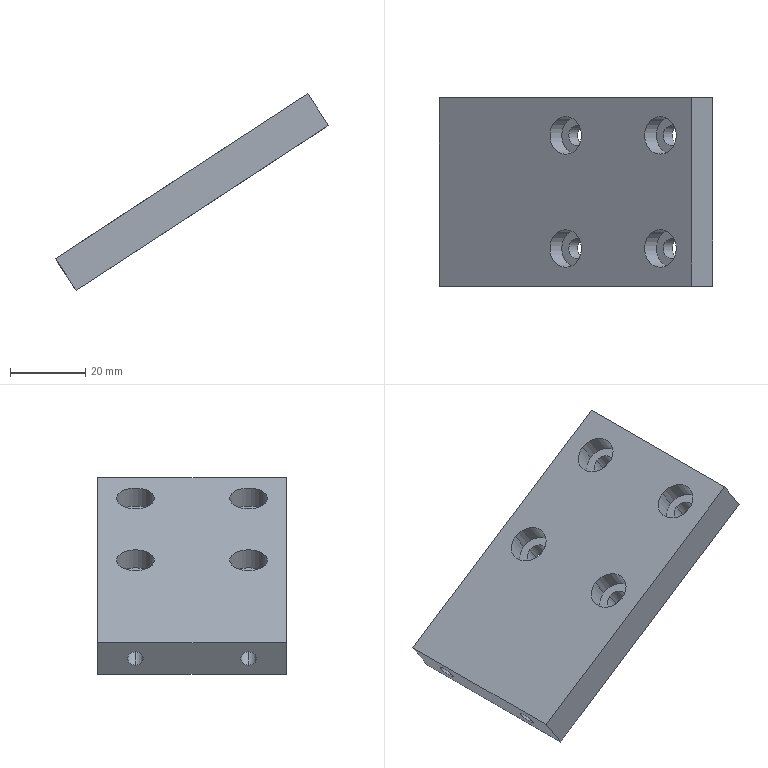Component | SolidWorks | ShimPlate02-1 | 1 solid | 34 faces | box 72.44 x 50 x 52.14 mm | volume 37445 mm3 | cylinder 20 | plane 10 | cone 4 | commonest cylinder face diameters 10 x8 5.5 x8 4.2 x4
build123d program:
from build123d import *

# Parameters (mm, degrees)
SKETCH1_W                                            = 50
SKETCH1_H                                            = 80
BOSS_EXTRUDE1_DEPTH                                  = 10
M5_TAPPED_HOLE1_D                                    = 4.2
M5_TAPPED_HOLE1_DEPTH                                = 12.4
M5_TAPPED_HOLE1_TIP                                  = 1.262
HOLE_SIZE_ACCORDING_TO_THE_TYPE_OF_HEXAG_D           = 5.5
HOLE_SIZE_ACCORDING_TO_THE_TYPE_OF_HEXAG_CBORE_D     = 10
HOLE_SIZE_ACCORDING_TO_THE_TYPE_OF_HEXAG_CBORE_DEPTH = 5.7


with BuildPart() as part:
    # Sketch1 → Boss-Extrude1 (new body)
    with BuildSketch(Plane.XY):
        Rectangle(SKETCH1_W, SKETCH1_H)
    extrude(amount=BOSS_EXTRUDE1_DEPTH)

    # M5 Tapped Hole1
    with Locations(Plane(origin=(0, -40, 0), x_dir=(-1, 0, 0), z_dir=(0, -1, 0))):
        with Locations((15, -5), (-15, -5)):
            Hole(M5_TAPPED_HOLE1_D / 2, depth=M5_TAPPED_HOLE1_DEPTH)
            with Locations((0, 0, -(M5_TAPPED_HOLE1_DEPTH + M5_TAPPED_HOLE1_TIP / 2))):  # 118° drill point
                Cone(0, M5_TAPPED_HOLE1_D / 2, M5_TAPPED_HOLE1_TIP, mode=Mode.SUBTRACT)

    # Hole Size according to the type of hexag (through all)
    with Locations(Plane.XY.offset(10)):
        with Locations((-15, 30), (15, 30), (15, 0), (-15, 0)):
            CounterBoreHole(HOLE_SIZE_ACCORDING_TO_THE_TYPE_OF_HEXAG_D / 2, HOLE_SIZE_ACCORDING_TO_THE_TYPE_OF_HEXAG_CBORE_D / 2, HOLE_SIZE_ACCORDING_TO_THE_TYPE_OF_HEXAG_CBORE_DEPTH)


solid = part.part

# Placed as in the assembly
solid = solid.moved(Location((-58.174, 149.546, 0.7149), (0, -33.165, -90)))
STEP:
#1=COLOUR_RGB('',0.7922,0.8196,0.9333);
#2=FILL_AREA_STYLE_COLOUR('',#1);
#3=FILL_AREA_STYLE('',(#2));
#4=SURFACE_STYLE_FILL_AREA(#3);
#5=SURFACE_SIDE_STYLE('',(#4));
#6=SURFACE_STYLE_USAGE(.BOTH.,#5);
#7=PRESENTATION_STYLE_ASSIGNMENT((#6));
#8=CARTESIAN_POINT('',(-1.394,6.675,0.816));
#9=VERTEX_POINT('',#8);
#10=CARTESIAN_POINT('',(-1.394,6.281,0.816));
#11=VERTEX_POINT('',#10);
#12=CARTESIAN_POINT('',(-1.394,6.478,0.816));
#13=DIRECTION('',(-0.5471,0.,0.8371));
#14=DIRECTION('',(-0.,-1.,0.));
#15=AXIS2_PLACEMENT_3D('',#12,#13,#14);
#16=CIRCLE('',#15,0.1969);
#17=EDGE_CURVE('',#9,#11,#16,.T.);
#18=ORIENTED_EDGE('',*,*,#17,.F.);
#19=CARTESIAN_POINT('',(-1.517,6.675,1.004));
#20=VERTEX_POINT('',#19);
#21=CARTESIAN_POINT('',(-1.517,6.675,1.004));
#22=DIRECTION('',(-0.5471,0.,0.8371));
#23=VECTOR('',#22,39.37);
#24=LINE('',#21,#23);
#25=EDGE_CURVE('',#9,#20,#24,.T.);
#26=ORIENTED_EDGE('',*,*,#25,.T.);
#27=CARTESIAN_POINT('',(-1.517,6.281,1.004));
#28=VERTEX_POINT('',#27);
#29=CARTESIAN_POINT('',(-1.517,6.478,1.004));
#30=DIRECTION('',(-0.5471,0.,0.8371));
#31=DIRECTION('',(-0.,-1.,0.));
#32=AXIS2_PLACEMENT_3D('',#29,#30,#31);
#33=CIRCLE('',#32,0.1969);
#34=EDGE_CURVE('',#20,#28,#33,.T.);
#35=ORIENTED_EDGE('',*,*,#34,.T.);
#36=CARTESIAN_POINT('',(-1.517,6.281,1.004));
#37=DIRECTION('',(-0.5471,0.,0.8371));
#38=VECTOR('',#37,39.37);
#39=LINE('',#36,#38);
#40=EDGE_CURVE('',#11,#28,#39,.T.);
#41=ORIENTED_EDGE('',*,*,#40,.F.);
#42=EDGE_LOOP('',(#18,#26,#35,#41));
#43=FACE_OUTER_BOUND('',#42,.T.);
#44=CARTESIAN_POINT('',(-1.517,6.478,1.004));
#45=DIRECTION('',(-0.5471,0.,0.8371));
#46=DIRECTION('',(-0.,-1.,0.));
#47=AXIS2_PLACEMENT_3D('',#44,#45,#46);
#48=CYLINDRICAL_SURFACE('',#47,0.1969);
#49=ADVANCED_FACE('',(#43),#48,.F.);
#50=CARTESIAN_POINT('',(-1.302,6.586,0.6743));
#51=VERTEX_POINT('',#50);
#52=CARTESIAN_POINT('',(-1.302,6.37,0.6743));
#53=VERTEX_POINT('',#52);
#54=CARTESIAN_POINT('',(-1.302,6.478,0.6743));
#55=DIRECTION('',(-0.5471,0.,0.8371));
#56=DIRECTION('',(0.,-1.,0.));
#57=AXIS2_PLACEMENT_3D('',#54,#55,#56);
#58=CIRCLE('',#57,0.1083);
#59=EDGE_CURVE('',#51,#53,#58,.T.);
#60=ORIENTED_EDGE('',*,*,#59,.F.);
#61=CARTESIAN_POINT('',(-1.394,6.586,0.816));
#62=VERTEX_POINT('',#61);
#63=CARTESIAN_POINT('',(-1.517,6.586,1.004));
#64=DIRECTION('',(-0.5471,0.,0.8371));
#65=VECTOR('',#64,39.37);
#66=LINE('',#63,#65);
#67=EDGE_CURVE('',#51,#62,#66,.T.);
#68=ORIENTED_EDGE('',*,*,#67,.T.);
#69=CARTESIAN_POINT('',(-1.394,6.37,0.816));
#70=VERTEX_POINT('',#69);
#71=CARTESIAN_POINT('',(-1.394,6.478,0.816));
#72=DIRECTION('',(-0.5471,0.,0.8371));
#73=DIRECTION('',(0.,-1.,0.));
#74=AXIS2_PLACEMENT_3D('',#71,#72,#73);
#75=CIRCLE('',#74,0.1083);
#76=EDGE_CURVE('',#62,#70,#75,.T.);
#77=ORIENTED_EDGE('',*,*,#76,.T.);
#78=CARTESIAN_POINT('',(-1.517,6.37,1.004));
#79=DIRECTION('',(-0.5471,0.,0.8371));
#80=VECTOR('',#79,39.37);
#81=LINE('',#78,#80);
#82=EDGE_CURVE('',#53,#70,#81,.T.);
#83=ORIENTED_EDGE('',*,*,#82,.F.);
#84=EDGE_LOOP('',(#60,#68,#77,#83));
#85=FACE_OUTER_BOUND('',#84,.T.);
#86=CARTESIAN_POINT('',(-1.517,6.478,1.004));
#87=DIRECTION('',(-0.5471,0.,0.8371));
#88=DIRECTION('',(0.,-1.,0.));
#89=AXIS2_PLACEMENT_3D('',#86,#87,#88);
#90=CYLINDRICAL_SURFACE('',#89,0.1083);
#91=ADVANCED_FACE('',(#85),#90,.F.);
#92=CARTESIAN_POINT('',(-1.394,5.494,0.816));
#93=VERTEX_POINT('',#92);
#94=CARTESIAN_POINT('',(-1.394,5.1,0.816));
#95=VERTEX_POINT('',#94);
#96=CARTESIAN_POINT('',(-1.394,5.297,0.816));
#97=DIRECTION('',(-0.5471,0.,0.8371));
#98=DIRECTION('',(-0.,-1.,0.));
#99=AXIS2_PLACEMENT_3D('',#96,#97,#98);
#100=CIRCLE('',#99,0.1969);
#101=EDGE_CURVE('',#93,#95,#100,.T.);
#102=ORIENTED_EDGE('',*,*,#101,.F.);
#103=CARTESIAN_POINT('',(-1.517,5.494,1.004));
#104=VERTEX_POINT('',#103);
#105=CARTESIAN_POINT('',(-1.517,5.494,1.004));
#106=DIRECTION('',(-0.5471,0.,0.8371));
#107=VECTOR('',#106,39.37);
#108=LINE('',#105,#107);
#109=EDGE_CURVE('',#93,#104,#108,.T.);
#110=ORIENTED_EDGE('',*,*,#109,.T.);
#111=CARTESIAN_POINT('',(-1.517,5.1,1.004));
#112=VERTEX_POINT('',#111);
#113=CARTESIAN_POINT('',(-1.517,5.297,1.004));
#114=DIRECTION('',(-0.5471,0.,0.8371));
#115=DIRECTION('',(-0.,-1.,0.));
#116=AXIS2_PLACEMENT_3D('',#113,#114,#115);
#117=CIRCLE('',#116,0.1969);
#118=EDGE_CURVE('',#104,#112,#117,.T.);
#119=ORIENTED_EDGE('',*,*,#118,.T.);
#120=CARTESIAN_POINT('',(-1.517,5.1,1.004));
#121=DIRECTION('',(-0.5471,0.,0.8371));
#122=VECTOR('',#121,39.37);
#123=LINE('',#120,#122);
#124=EDGE_CURVE('',#95,#112,#123,.T.);
#125=ORIENTED_EDGE('',*,*,#124,.F.);
#126=EDGE_LOOP('',(#102,#110,#119,#125));
#127=FACE_OUTER_BOUND('',#126,.T.);
#128=CARTESIAN_POINT('',(-1.517,5.297,1.004));
#129=DIRECTION('',(-0.5471,0.,0.8371));
#130=DIRECTION('',(-0.,-1.,0.));
#131=AXIS2_PLACEMENT_3D('',#128,#129,#130);
#132=CYLINDRICAL_SURFACE('',#131,0.1969);
#133=ADVANCED_FACE('',(#127),#132,.F.);
#134=CARTESIAN_POINT('',(-1.302,5.405,0.6743));
#135=VERTEX_POINT('',#134);
#136=CARTESIAN_POINT('',(-1.302,5.189,0.6743));
#137=VERTEX_POINT('',#136);
#138=CARTESIAN_POINT('',(-1.302,5.297,0.6743));
#139=DIRECTION('',(-0.5471,0.,0.8371));
#140=DIRECTION('',(0.,-1.,0.));
#141=AXIS2_PLACEMENT_3D('',#138,#139,#140);
#142=CIRCLE('',#141,0.1083);
#143=EDGE_CURVE('',#135,#137,#142,.T.);
#144=ORIENTED_EDGE('',*,*,#143,.F.);
#145=CARTESIAN_POINT('',(-1.394,5.405,0.816));
#146=VERTEX_POINT('',#145);
#147=CARTESIAN_POINT('',(-1.517,5.405,1.004));
#148=DIRECTION('',(-0.5471,0.,0.8371));
#149=VECTOR('',#148,39.37);
#150=LINE('',#147,#149);
#151=EDGE_CURVE('',#135,#146,#150,.T.);
#152=ORIENTED_EDGE('',*,*,#151,.T.);
#153=CARTESIAN_POINT('',(-1.394,5.189,0.816));
#154=VERTEX_POINT('',#153);
#155=CARTESIAN_POINT('',(-1.394,5.297,0.816));
#156=DIRECTION('',(-0.5471,0.,0.8371));
#157=DIRECTION('',(0.,-1.,0.));
#158=AXIS2_PLACEMENT_3D('',#155,#156,#157);
#159=CIRCLE('',#158,0.1083);
#160=EDGE_CURVE('',#146,#154,#159,.T.);
#161=ORIENTED_EDGE('',*,*,#160,.T.);
#162=CARTESIAN_POINT('',(-1.517,5.189,1.004));
#163=DIRECTION('',(-0.5471,0.,0.8371));
#164=VECTOR('',#163,39.37);
#165=LINE('',#162,#164);
#166=EDGE_CURVE('',#137,#154,#165,.T.);
#167=ORIENTED_EDGE('',*,*,#166,.F.);
#168=EDGE_LOOP('',(#144,#152,#161,#167));
#169=FACE_OUTER_BOUND('',#168,.T.);
#170=CARTESIAN_POINT('',(-1.517,5.297,1.004));
#171=DIRECTION('',(-0.5471,0.,0.8371));
#172=DIRECTION('',(0.,-1.,0.));
#173=AXIS2_PLACEMENT_3D('',#170,#171,#172);
#174=CYLINDRICAL_SURFACE('',#173,0.1083);
#175=ADVANCED_FACE('',(#169),#174,.F.);
#176=CARTESIAN_POINT('',(-2.383,5.494,0.1699));
#177=VERTEX_POINT('',#176);
#178=CARTESIAN_POINT('',(-2.383,5.1,0.1699));
#179=VERTEX_POINT('',#178);
#180=CARTESIAN_POINT('',(-2.383,5.297,0.1699));
#181=DIRECTION('',(-0.5471,0.,0.8371));
#182=DIRECTION('',(-0.,-1.,0.));
#183=AXIS2_PLACEMENT_3D('',#180,#181,#182);
#184=CIRCLE('',#183,0.1969);
#185=EDGE_CURVE('',#177,#179,#184,.T.);
#186=ORIENTED_EDGE('',*,*,#185,.F.);
#187=CARTESIAN_POINT('',(-2.506,5.494,0.3577));
#188=VERTEX_POINT('',#187);
#189=CARTESIAN_POINT('',(-2.506,5.494,0.3577));
#190=DIRECTION('',(-0.5471,0.,0.8371));
#191=VECTOR('',#190,39.37);
#192=LINE('',#189,#191);
#193=EDGE_CURVE('',#177,#188,#192,.T.);
#194=ORIENTED_EDGE('',*,*,#193,.T.);
#195=CARTESIAN_POINT('',(-2.506,5.1,0.3577));
#196=VERTEX_POINT('',#195);
#197=CARTESIAN_POINT('',(-2.506,5.297,0.3577));
#198=DIRECTION('',(-0.5471,0.,0.8371));
#199=DIRECTION('',(0.,-1.,0.));
#200=AXIS2_PLACEMENT_3D('',#197,#198,#199);
#201=CIRCLE('',#200,0.1969);
#202=EDGE_CURVE('',#188,#196,#201,.T.);
#203=ORIENTED_EDGE('',*,*,#202,.T.);
#204=CARTESIAN_POINT('',(-2.506,5.1,0.3577));
#205=DIRECTION('',(-0.5471,0.,0.8371));
#206=VECTOR('',#205,39.37);
#207=LINE('',#204,#206);
#208=EDGE_CURVE('',#179,#196,#207,.T.);
#209=ORIENTED_EDGE('',*,*,#208,.F.);
#210=EDGE_LOOP('',(#186,#194,#203,#209));
#211=FACE_OUTER_BOUND('',#210,.T.);
#212=CARTESIAN_POINT('',(-2.506,5.297,0.3577));
#213=DIRECTION('',(-0.5471,0.,0.8371));
#214=DIRECTION('',(0.,-1.,0.));
#215=AXIS2_PLACEMENT_3D('',#212,#213,#214);
#216=CYLINDRICAL_SURFACE('',#215,0.1969);
#217=ADVANCED_FACE('',(#211),#216,.F.);
#218=CARTESIAN_POINT('',(-2.29,5.405,0.02814));
#219=VERTEX_POINT('',#218);
#220=CARTESIAN_POINT('',(-2.29,5.189,0.02814));
#221=VERTEX_POINT('',#220);
#222=CARTESIAN_POINT('',(-2.29,5.297,0.02814));
#223=DIRECTION('',(-0.5471,0.,0.8371));
#224=DIRECTION('',(0.,-1.,0.));
#225=AXIS2_PLACEMENT_3D('',#222,#223,#224);
#226=CIRCLE('',#225,0.1083);
#227=EDGE_CURVE('',#219,#221,#226,.T.);
#228=ORIENTED_EDGE('',*,*,#227,.F.);
#229=CARTESIAN_POINT('',(-2.383,5.405,0.1699));
#230=VERTEX_POINT('',#229);
#231=CARTESIAN_POINT('',(-2.506,5.405,0.3577));
#232=DIRECTION('',(-0.5471,0.,0.8371));
#233=VECTOR('',#232,39.37);
#234=LINE('',#231,#233);
#235=EDGE_CURVE('',#219,#230,#234,.T.);
#236=ORIENTED_EDGE('',*,*,#235,.T.);
#237=CARTESIAN_POINT('',(-2.383,5.189,0.1699));
#238=VERTEX_POINT('',#237);
#239=CARTESIAN_POINT('',(-2.383,5.297,0.1699));
#240=DIRECTION('',(-0.5471,0.,0.8371));
#241=DIRECTION('',(0.,-1.,0.));
#242=AXIS2_PLACEMENT_3D('',#239,#240,#241);
#243=CIRCLE('',#242,0.1083);
#244=EDGE_CURVE('',#230,#238,#243,.T.);
#245=ORIENTED_EDGE('',*,*,#244,.T.);
#246=CARTESIAN_POINT('',(-2.506,5.189,0.3577));
#247=DIRECTION('',(-0.5471,0.,0.8371));
#248=VECTOR('',#247,39.37);
#249=LINE('',#246,#248);
#250=EDGE_CURVE('',#221,#238,#249,.T.);
#251=ORIENTED_EDGE('',*,*,#250,.F.);
#252=EDGE_LOOP('',(#228,#236,#245,#251));
#253=FACE_OUTER_BOUND('',#252,.T.);
#254=CARTESIAN_POINT('',(-2.506,5.297,0.3577));
#255=DIRECTION('',(-0.5471,0.,0.8371));
#256=DIRECTION('',(0.,-1.,0.));
#257=AXIS2_PLACEMENT_3D('',#254,#255,#256);
#258=CYLINDRICAL_SURFACE('',#257,0.1083);
#259=ADVANCED_FACE('',(#253),#258,.F.);
#260=CARTESIAN_POINT('',(-2.383,6.675,0.1699));
#261=VERTEX_POINT('',#260);
#262=CARTESIAN_POINT('',(-2.383,6.281,0.1699));
#263=VERTEX_POINT('',#262);
#264=CARTESIAN_POINT('',(-2.383,6.478,0.1699));
#265=DIRECTION('',(-0.5471,0.,0.8371));
#266=DIRECTION('',(-0.,-1.,0.));
#267=AXIS2_PLACEMENT_3D('',#264,#265,#266);
#268=CIRCLE('',#267,0.1969);
#269=EDGE_CURVE('',#261,#263,#268,.T.);
#270=ORIENTED_EDGE('',*,*,#269,.F.);
#271=CARTESIAN_POINT('',(-2.506,6.675,0.3577));
#272=VERTEX_POINT('',#271);
#273=CARTESIAN_POINT('',(-2.506,6.675,0.3577));
#274=DIRECTION('',(-0.5471,0.,0.8371));
#275=VECTOR('',#274,39.37);
#276=LINE('',#273,#275);
#277=EDGE_CURVE('',#261,#272,#276,.T.);
#278=ORIENTED_EDGE('',*,*,#277,.T.);
#279=CARTESIAN_POINT('',(-2.506,6.281,0.3577));
#280=VERTEX_POINT('',#279);
#281=CARTESIAN_POINT('',(-2.506,6.478,0.3577));
#282=DIRECTION('',(-0.5471,0.,0.8371));
#283=DIRECTION('',(0.,-1.,0.));
#284=AXIS2_PLACEMENT_3D('',#281,#282,#283);
#285=CIRCLE('',#284,0.1969);
#286=EDGE_CURVE('',#272,#280,#285,.T.);
#287=ORIENTED_EDGE('',*,*,#286,.T.);
#288=CARTESIAN_POINT('',(-2.506,6.281,0.3577));
#289=DIRECTION('',(-0.5471,0.,0.8371));
#290=VECTOR('',#289,39.37);
#291=LINE('',#288,#290);
#292=EDGE_CURVE('',#263,#280,#291,.T.);
#293=ORIENTED_EDGE('',*,*,#292,.F.);
#294=EDGE_LOOP('',(#270,#278,#287,#293));
#295=FACE_OUTER_BOUND('',#294,.T.);
#296=CARTESIAN_POINT('',(-2.506,6.478,0.3577));
#297=DIRECTION('',(-0.5471,0.,0.8371));
#298=DIRECTION('',(0.,-1.,0.));
#299=AXIS2_PLACEMENT_3D('',#296,#297,#298);
#300=CYLINDRICAL_SURFACE('',#299,0.1969);
#301=ADVANCED_FACE('',(#295),#300,.F.);
#302=CARTESIAN_POINT('',(-2.29,6.586,0.02814));
#303=VERTEX_POINT('',#302);
#304=CARTESIAN_POINT('',(-2.29,6.37,0.02814));
#305=VERTEX_POINT('',#304);
#306=CARTESIAN_POINT('',(-2.29,6.478,0.02814));
#307=DIRECTION('',(-0.5471,0.,0.8371));
#308=DIRECTION('',(0.,-1.,0.));
#309=AXIS2_PLACEMENT_3D('',#306,#307,#308);
#310=CIRCLE('',#309,0.1083);
#311=EDGE_CURVE('',#303,#305,#310,.T.);
#312=ORIENTED_EDGE('',*,*,#311,.F.);
#313=CARTESIAN_POINT('',(-2.383,6.586,0.1699));
#314=VERTEX_POINT('',#313);
#315=CARTESIAN_POINT('',(-2.506,6.586,0.3577));
#316=DIRECTION('',(-0.5471,0.,0.8371));
#317=VECTOR('',#316,39.37);
#318=LINE('',#315,#317);
#319=EDGE_CURVE('',#303,#314,#318,.T.);
#320=ORIENTED_EDGE('',*,*,#319,.T.);
#321=CARTESIAN_POINT('',(-2.383,6.37,0.1699));
#322=VERTEX_POINT('',#321);
#323=CARTESIAN_POINT('',(-2.383,6.478,0.1699));
#324=DIRECTION('',(-0.5471,0.,0.8371));
#325=DIRECTION('',(0.,-1.,0.));
#326=AXIS2_PLACEMENT_3D('',#323,#324,#325);
#327=CIRCLE('',#326,0.1083);
#328=EDGE_CURVE('',#314,#322,#327,.T.);
#329=ORIENTED_EDGE('',*,*,#328,.T.);
#330=CARTESIAN_POINT('',(-2.506,6.37,0.3577));
#331=DIRECTION('',(-0.5471,0.,0.8371));
#332=VECTOR('',#331,39.37);
#333=LINE('',#330,#332);
#334=EDGE_CURVE('',#305,#322,#333,.T.);
#335=ORIENTED_EDGE('',*,*,#334,.F.);
#336=EDGE_LOOP('',(#312,#320,#329,#335));
#337=FACE_OUTER_BOUND('',#336,.T.);
#338=CARTESIAN_POINT('',(-2.506,6.478,0.3577));
#339=DIRECTION('',(-0.5471,0.,0.8371));
#340=DIRECTION('',(0.,-1.,0.));
#341=AXIS2_PLACEMENT_3D('',#338,#339,#340);
#342=CYLINDRICAL_SURFACE('',#341,0.1083);
#343=ADVANCED_FACE('',(#337),#342,.F.);
#344=CARTESIAN_POINT('',(-3.353,6.478,-0.3323));
#345=VERTEX_POINT('',#344);
#346=CARTESIAN_POINT('',(-3.262,6.478,-0.4707));
#347=VERTEX_POINT('',#346);
#348=CARTESIAN_POINT('',(-3.308,6.478,-0.4015));
#349=DIRECTION('',(-0.8371,-0.,-0.5471));
#350=DIRECTION('',(0.5471,0.,-0.8371));
#351=AXIS2_PLACEMENT_3D('',#348,#349,#350);
#352=CIRCLE('',#351,0.08268);
#353=EDGE_CURVE('',#345,#347,#352,.T.);
#354=ORIENTED_EDGE('',*,*,#353,.F.);
#355=CARTESIAN_POINT('',(-3.762,6.478,-0.5994));
#356=VERTEX_POINT('',#355);
#357=CARTESIAN_POINT('',(-3.762,6.478,-0.5994));
#358=DIRECTION('',(-0.8371,-0.,-0.5471));
#359=VECTOR('',#358,39.37);
#360=LINE('',#357,#359);
#361=EDGE_CURVE('',#345,#356,#360,.T.);
#362=ORIENTED_EDGE('',*,*,#361,.T.);
#363=CARTESIAN_POINT('',(-3.671,6.478,-0.7378));
#364=VERTEX_POINT('',#363);
#365=CARTESIAN_POINT('',(-3.716,6.478,-0.6686));
#366=DIRECTION('',(-0.8371,-0.,-0.5471));
#367=DIRECTION('',(0.5471,0.,-0.8371));
#368=AXIS2_PLACEMENT_3D('',#365,#366,#367);
#369=CIRCLE('',#368,0.08268);
#370=EDGE_CURVE('',#356,#364,#369,.T.);
#371=ORIENTED_EDGE('',*,*,#370,.T.);
#372=CARTESIAN_POINT('',(-3.671,6.478,-0.7378));
#373=DIRECTION('',(-0.8371,-0.,-0.5471));
#374=VECTOR('',#373,39.37);
#375=LINE('',#372,#374);
#376=EDGE_CURVE('',#347,#364,#375,.T.);
#377=ORIENTED_EDGE('',*,*,#376,.F.);
#378=EDGE_LOOP('',(#354,#362,#371,#377));
#379=FACE_OUTER_BOUND('',#378,.T.);
#380=CARTESIAN_POINT('',(-3.716,6.478,-0.6686));
#381=DIRECTION('',(-0.8371,-0.,-0.5471));
#382=DIRECTION('',(0.5471,0.,-0.8371));
#383=AXIS2_PLACEMENT_3D('',#380,#381,#382);
#384=CYLINDRICAL_SURFACE('',#383,0.08268);
#385=ADVANCED_FACE('',(#379),#384,.F.);
#386=CARTESIAN_POINT('',(-3.266,6.478,-0.3743));
#387=VERTEX_POINT('',#386);
#388=CARTESIAN_POINT('',(-3.262,6.478,-0.4707));
#389=DIRECTION('',(0.03778,-0.,-0.9993));
#390=VECTOR('',#389,39.37);
#391=LINE('',#388,#390);
#392=EDGE_CURVE('',#387,#347,#391,.T.);
#393=ORIENTED_EDGE('',*,*,#392,.F.);
#394=CARTESIAN_POINT('',(-3.353,6.478,-0.3323));
#395=DIRECTION('',(-0.9001,0.,0.4358));
#396=VECTOR('',#395,39.37);
#397=LINE('',#394,#396);
#398=EDGE_CURVE('',#387,#345,#397,.T.);
#399=ORIENTED_EDGE('',*,*,#398,.T.);
#400=ORIENTED_EDGE('',*,*,#353,.T.);
#401=EDGE_LOOP('',(#393,#399,#400));
#402=FACE_OUTER_BOUND('',#401,.T.);
#403=CARTESIAN_POINT('',(-3.308,6.478,-0.4015));
#404=DIRECTION('',(-0.8371,-0.,-0.5471));
#405=DIRECTION('',(0.5471,0.,-0.8371));
#406=AXIS2_PLACEMENT_3D('',#403,#404,#405);
#407=CONICAL_SURFACE('',#406,0.08268,1.03);
#408=ADVANCED_FACE('',(#402),#407,.F.);
#409=CARTESIAN_POINT('',(-3.353,5.297,-0.3323));
#410=VERTEX_POINT('',#409);
#411=CARTESIAN_POINT('',(-3.262,5.297,-0.4707));
#412=VERTEX_POINT('',#411);
#413=CARTESIAN_POINT('',(-3.308,5.297,-0.4015));
#414=DIRECTION('',(-0.8371,-0.,-0.5471));
#415=DIRECTION('',(0.5471,0.,-0.8371));
#416=AXIS2_PLACEMENT_3D('',#413,#414,#415);
#417=CIRCLE('',#416,0.08268);
#418=EDGE_CURVE('',#410,#412,#417,.T.);
#419=ORIENTED_EDGE('',*,*,#418,.F.);
#420=CARTESIAN_POINT('',(-3.762,5.297,-0.5994));
#421=VERTEX_POINT('',#420);
#422=CARTESIAN_POINT('',(-3.762,5.297,-0.5994));
#423=DIRECTION('',(-0.8371,-0.,-0.5471));
#424=VECTOR('',#423,39.37);
#425=LINE('',#422,#424);
#426=EDGE_CURVE('',#410,#421,#425,.T.);
#427=ORIENTED_EDGE('',*,*,#426,.T.);
#428=CARTESIAN_POINT('',(-3.671,5.297,-0.7378));
#429=VERTEX_POINT('',#428);
#430=CARTESIAN_POINT('',(-3.716,5.297,-0.6686));
#431=DIRECTION('',(-0.8371,-0.,-0.5471));
#432=DIRECTION('',(0.5471,0.,-0.8371));
#433=AXIS2_PLACEMENT_3D('',#430,#431,#432);
#434=CIRCLE('',#433,0.08268);
#435=EDGE_CURVE('',#421,#429,#434,.T.);
#436=ORIENTED_EDGE('',*,*,#435,.T.);
#437=CARTESIAN_POINT('',(-3.671,5.297,-0.7378));
#438=DIRECTION('',(-0.8371,-0.,-0.5471));
#439=VECTOR('',#438,39.37);
#440=LINE('',#437,#439);
#441=EDGE_CURVE('',#412,#429,#440,.T.);
#442=ORIENTED_EDGE('',*,*,#441,.F.);
#443=EDGE_LOOP('',(#419,#427,#436,#442));
#444=FACE_OUTER_BOUND('',#443,.T.);
#445=CARTESIAN_POINT('',(-3.716,5.297,-0.6686));
#446=DIRECTION('',(-0.8371,-0.,-0.5471));
#447=DIRECTION('',(0.5471,0.,-0.8371));
#448=AXIS2_PLACEMENT_3D('',#445,#446,#447);
#449=CYLINDRICAL_SURFACE('',#448,0.08268);
#450=ADVANCED_FACE('',(#444),#449,.F.);
#451=CARTESIAN_POINT('',(-3.266,5.297,-0.3743));
#452=VERTEX_POINT('',#451);
#453=CARTESIAN_POINT('',(-3.262,5.297,-0.4707));
#454=DIRECTION('',(0.03778,-0.,-0.9993));
#455=VECTOR('',#454,39.37);
#456=LINE('',#453,#455);
#457=EDGE_CURVE('',#452,#412,#456,.T.);
#458=ORIENTED_EDGE('',*,*,#457,.F.);
#459=CARTESIAN_POINT('',(-3.353,5.297,-0.3323));
#460=DIRECTION('',(-0.9001,0.,0.4358));
#461=VECTOR('',#460,39.37);
#462=LINE('',#459,#461);
#463=EDGE_CURVE('',#452,#410,#462,.T.);
#464=ORIENTED_EDGE('',*,*,#463,.T.);
#465=ORIENTED_EDGE('',*,*,#418,.T.);
#466=EDGE_LOOP('',(#458,#464,#465));
#467=FACE_OUTER_BOUND('',#466,.T.);
#468=CARTESIAN_POINT('',(-3.308,5.297,-0.4015));
#469=DIRECTION('',(-0.8371,-0.,-0.5471));
#470=DIRECTION('',(0.5471,0.,-0.8371));
#471=AXIS2_PLACEMENT_3D('',#468,#469,#470);
#472=CONICAL_SURFACE('',#471,0.08268,1.03);
#473=ADVANCED_FACE('',(#467),#472,.F.);
#474=CARTESIAN_POINT('',(-3.609,4.903,-0.8334));
#475=VERTEX_POINT('',#474);
#476=CARTESIAN_POINT('',(-0.9721,4.903,0.8896));
#477=VERTEX_POINT('',#476);
#478=CARTESIAN_POINT('',(-3.609,4.903,-0.8334));
#479=DIRECTION('',(0.8371,0.,0.5471));
#480=VECTOR('',#479,39.37);
#481=LINE('',#478,#480);
#482=EDGE_CURVE('',#475,#477,#481,.T.);
#483=ORIENTED_EDGE('',*,*,#482,.T.);
#484=CARTESIAN_POINT('',(-1.187,4.903,1.219));
#485=VERTEX_POINT('',#484);
#486=CARTESIAN_POINT('',(-1.187,4.903,1.219));
#487=DIRECTION('',(0.5471,-0.,-0.8371));
#488=VECTOR('',#487,39.37);
#489=LINE('',#486,#488);
#490=EDGE_CURVE('',#485,#477,#489,.T.);
#491=ORIENTED_EDGE('',*,*,#490,.F.);
#492=CARTESIAN_POINT('',(-3.824,4.903,-0.5038));
#493=VERTEX_POINT('',#492);
#494=CARTESIAN_POINT('',(-3.824,4.903,-0.5038));
#495=DIRECTION('',(0.8371,0.,0.5471));
#496=VECTOR('',#495,39.37);
#497=LINE('',#494,#496);
#498=EDGE_CURVE('',#493,#485,#497,.T.);
#499=ORIENTED_EDGE('',*,*,#498,.F.);
#500=CARTESIAN_POINT('',(-3.824,4.903,-0.5038));
#501=DIRECTION('',(0.5471,-0.,-0.8371));
#502=VECTOR('',#501,39.37);
#503=LINE('',#500,#502);
#504=EDGE_CURVE('',#493,#475,#503,.T.);
#505=ORIENTED_EDGE('',*,*,#504,.T.);
#506=EDGE_LOOP('',(#483,#491,#499,#505));
#507=FACE_OUTER_BOUND('',#506,.T.);
#508=CARTESIAN_POINT('',(-3.824,4.903,-0.5038));
#509=DIRECTION('',(0.,1.,-0.));
#510=DIRECTION('',(-0.5471,0.,0.8371));
#511=AXIS2_PLACEMENT_3D('',#508,#509,#510);
#512=PLANE('',#511);
#513=ADVANCED_FACE('',(#507),#512,.F.);
#514=CARTESIAN_POINT('',(-0.9721,6.872,0.8896));
#515=VERTEX_POINT('',#514);
#516=CARTESIAN_POINT('',(-0.9721,6.872,0.8896));
#517=DIRECTION('',(0.,1.,-0.));
#518=VECTOR('',#517,39.37);
#519=LINE('',#516,#518);
#520=EDGE_CURVE('',#477,#515,#519,.T.);
#521=ORIENTED_EDGE('',*,*,#520,.T.);
#522=CARTESIAN_POINT('',(-1.187,6.872,1.219));
#523=VERTEX_POINT('',#522);
#524=CARTESIAN_POINT('',(-1.187,6.872,1.219));
#525=DIRECTION('',(0.5471,-0.,-0.8371));
#526=VECTOR('',#525,39.37);
#527=LINE('',#524,#526);
#528=EDGE_CURVE('',#523,#515,#527,.T.);
#529=ORIENTED_EDGE('',*,*,#528,.F.);
#530=CARTESIAN_POINT('',(-1.187,6.872,1.219));
#531=DIRECTION('',(0.,1.,-0.));
#532=VECTOR('',#531,39.37);
#533=LINE('',#530,#532);
#534=EDGE_CURVE('',#485,#523,#533,.T.);
#535=ORIENTED_EDGE('',*,*,#534,.F.);
#536=ORIENTED_EDGE('',*,*,#490,.T.);
#537=EDGE_LOOP('',(#521,#529,#535,#536));
#538=FACE_OUTER_BOUND('',#537,.T.);
#539=CARTESIAN_POINT('',(-1.187,6.872,1.219));
#540=DIRECTION('',(-0.8371,-0.,-0.5471));
#541=DIRECTION('',(0.5471,-0.,-0.8371));
#542=AXIS2_PLACEMENT_3D('',#539,#540,#541);
#543=PLANE('',#542);
#544=ADVANCED_FACE('',(#538),#543,.F.);
#545=CARTESIAN_POINT('',(-3.609,6.872,-0.8334));
#546=VERTEX_POINT('',#545);
#547=CARTESIAN_POINT('',(-3.609,6.872,-0.8334));
#548=DIRECTION('',(-0.8371,-0.,-0.5471));
#549=VECTOR('',#548,39.37);
#550=LINE('',#547,#549);
#551=EDGE_CURVE('',#515,#546,#550,.T.);
#552=ORIENTED_EDGE('',*,*,#551,.T.);
#553=CARTESIAN_POINT('',(-3.824,6.872,-0.5038));
#554=VERTEX_POINT('',#553);
#555=CARTESIAN_POINT('',(-3.824,6.872,-0.5038));
#556=DIRECTION('',(0.5471,-0.,-0.8371));
#557=VECTOR('',#556,39.37);
#558=LINE('',#555,#557);
#559=EDGE_CURVE('',#554,#546,#558,.T.);
#560=ORIENTED_EDGE('',*,*,#559,.F.);
#561=CARTESIAN_POINT('',(-3.824,6.872,-0.5038));
#562=DIRECTION('',(-0.8371,-0.,-0.5471));
#563=VECTOR('',#562,39.37);
#564=LINE('',#561,#563);
#565=EDGE_CURVE('',#523,#554,#564,.T.);
#566=ORIENTED_EDGE('',*,*,#565,.F.);
#567=ORIENTED_EDGE('',*,*,#528,.T.);
#568=EDGE_LOOP('',(#552,#560,#566,#567));
#569=FACE_OUTER_BOUND('',#568,.T.);
#570=CARTESIAN_POINT('',(-3.824,6.872,-0.5038));
#571=DIRECTION('',(-0.,-1.,0.));
#572=DIRECTION('',(0.5471,-0.,-0.8371));
#573=AXIS2_PLACEMENT_3D('',#570,#571,#572);
#574=PLANE('',#573);
#575=ADVANCED_FACE('',(#569),#574,.F.);
#576=CARTESIAN_POINT('',(-3.716,6.478,-0.6686));
#577=DIRECTION('',(-0.8371,-0.,-0.5471));
#578=DIRECTION('',(0.5471,0.,-0.8371));
#579=AXIS2_PLACEMENT_3D('',#576,#577,#578);
#580=CIRCLE('',#579,0.08268);
#581=EDGE_CURVE('',#364,#356,#580,.T.);
#582=ORIENTED_EDGE('',*,*,#581,.F.);
#583=ORIENTED_EDGE('',*,*,#370,.F.);
#584=EDGE_LOOP('',(#582,#583));
#585=FACE_BOUND('',#584,.T.);
#586=CARTESIAN_POINT('',(-3.716,5.297,-0.6686));
#587=DIRECTION('',(-0.8371,-0.,-0.5471));
#588=DIRECTION('',(0.5471,0.,-0.8371));
#589=AXIS2_PLACEMENT_3D('',#586,#587,#588);
#590=CIRCLE('',#589,0.08268);
#591=EDGE_CURVE('',#429,#421,#590,.T.);
#592=ORIENTED_EDGE('',*,*,#591,.F.);
#593=ORIENTED_EDGE('',*,*,#435,.F.);
#594=EDGE_LOOP('',(#592,#593));
#595=FACE_BOUND('',#594,.T.);
#596=CARTESIAN_POINT('',(-3.609,6.872,-0.8334));
#597=DIRECTION('',(-0.,-1.,0.));
#598=VECTOR('',#597,39.37);
#599=LINE('',#596,#598);
#600=EDGE_CURVE('',#546,#475,#599,.T.);
#601=ORIENTED_EDGE('',*,*,#600,.T.);
#602=ORIENTED_EDGE('',*,*,#504,.F.);
#603=CARTESIAN_POINT('',(-3.824,6.872,-0.5038));
#604=DIRECTION('',(-0.,-1.,0.));
#605=VECTOR('',#604,39.37);
#606=LINE('',#603,#605);
#607=EDGE_CURVE('',#554,#493,#606,.T.);
#608=ORIENTED_EDGE('',*,*,#607,.F.);
#609=ORIENTED_EDGE('',*,*,#559,.T.);
#610=EDGE_LOOP('',(#601,#602,#608,#609));
#611=FACE_OUTER_BOUND('',#610,.T.);
#612=CARTESIAN_POINT('',(-3.824,6.872,-0.5038));
#613=DIRECTION('',(0.8371,0.,0.5471));
#614=DIRECTION('',(-0.5471,0.,0.8371));
#615=AXIS2_PLACEMENT_3D('',#612,#613,#614);
#616=PLANE('',#615);
#617=ADVANCED_FACE('',(#585,#595,#611),#616,.F.);
#618=CARTESIAN_POINT('',(-1.517,6.478,1.004));
#619=DIRECTION('',(-0.5471,0.,0.8371));
#620=DIRECTION('',(-0.,-1.,0.));
#621=AXIS2_PLACEMENT_3D('',#618,#619,#620);
#622=CIRCLE('',#621,0.1969);
#623=EDGE_CURVE('',#28,#20,#622,.T.);
#624=ORIENTED_EDGE('',*,*,#623,.F.);
#625=ORIENTED_EDGE('',*,*,#34,.F.);
#626=EDGE_LOOP('',(#624,#625));
#627=FACE_BOUND('',#626,.T.);
#628=CARTESIAN_POINT('',(-1.517,5.297,1.004));
#629=DIRECTION('',(-0.5471,0.,0.8371));
#630=DIRECTION('',(-0.,-1.,0.));
#631=AXIS2_PLACEMENT_3D('',#628,#629,#630);
#632=CIRCLE('',#631,0.1969);
#633=EDGE_CURVE('',#112,#104,#632,.T.);
#634=ORIENTED_EDGE('',*,*,#633,.F.);
#635=ORIENTED_EDGE('',*,*,#118,.F.);
#636=EDGE_LOOP('',(#634,#635));
#637=FACE_BOUND('',#636,.T.);
#638=CARTESIAN_POINT('',(-2.506,5.297,0.3577));
#639=DIRECTION('',(-0.5471,0.,0.8371));
#640=DIRECTION('',(0.,-1.,0.));
#641=AXIS2_PLACEMENT_3D('',#638,#639,#640);
#642=CIRCLE('',#641,0.1969);
#643=EDGE_CURVE('',#196,#188,#642,.T.);
#644=ORIENTED_EDGE('',*,*,#643,.F.);
#645=ORIENTED_EDGE('',*,*,#202,.F.);
#646=EDGE_LOOP('',(#644,#645));
#647=FACE_BOUND('',#646,.T.);
#648=CARTESIAN_POINT('',(-2.506,6.478,0.3577));
#649=DIRECTION('',(-0.5471,0.,0.8371));
#650=DIRECTION('',(0.,-1.,0.));
#651=AXIS2_PLACEMENT_3D('',#648,#649,#650);
#652=CIRCLE('',#651,0.1969);
#653=EDGE_CURVE('',#280,#272,#652,.T.);
#654=ORIENTED_EDGE('',*,*,#653,.F.);
#655=ORIENTED_EDGE('',*,*,#286,.F.);
#656=EDGE_LOOP('',(#654,#655));
#657=FACE_BOUND('',#656,.T.);
#658=ORIENTED_EDGE('',*,*,#498,.T.);
#659=ORIENTED_EDGE('',*,*,#534,.T.);
#660=ORIENTED_EDGE('',*,*,#565,.T.);
#661=ORIENTED_EDGE('',*,*,#607,.T.);
#662=EDGE_LOOP('',(#658,#659,#660,#661));
#663=FACE_OUTER_BOUND('',#662,.T.);
#664=CARTESIAN_POINT('',(-2.506,5.888,0.3577));
#665=DIRECTION('',(0.5471,-0.,-0.8371));
#666=DIRECTION('',(0.,1.,-0.));
#667=AXIS2_PLACEMENT_3D('',#664,#665,#666);
#668=PLANE('',#667);
#669=ADVANCED_FACE('',(#627,#637,#647,#657,#663),#668,.F.);
#670=CARTESIAN_POINT('',(-1.302,6.478,0.6743));
#671=DIRECTION('',(-0.5471,0.,0.8371));
#672=DIRECTION('',(0.,-1.,0.));
#673=AXIS2_PLACEMENT_3D('',#670,#671,#672);
#674=CIRCLE('',#673,0.1083);
#675=EDGE_CURVE('',#53,#51,#674,.T.);
#676=ORIENTED_EDGE('',*,*,#675,.T.);
#677=ORIENTED_EDGE('',*,*,#59,.T.);
#678=EDGE_LOOP('',(#676,#677));
#679=FACE_BOUND('',#678,.T.);
#680=CARTESIAN_POINT('',(-1.302,5.297,0.6743));
#681=DIRECTION('',(-0.5471,0.,0.8371));
#682=DIRECTION('',(0.,-1.,0.));
#683=AXIS2_PLACEMENT_3D('',#680,#681,#682);
#684=CIRCLE('',#683,0.1083);
#685=EDGE_CURVE('',#137,#135,#684,.T.);
#686=ORIENTED_EDGE('',*,*,#685,.T.);
#687=ORIENTED_EDGE('',*,*,#143,.T.);
#688=EDGE_LOOP('',(#686,#687));
#689=FACE_BOUND('',#688,.T.);
#690=CARTESIAN_POINT('',(-2.29,5.297,0.02814));
#691=DIRECTION('',(-0.5471,0.,0.8371));
#692=DIRECTION('',(0.,-1.,0.));
#693=AXIS2_PLACEMENT_3D('',#690,#691,#692);
#694=CIRCLE('',#693,0.1083);
#695=EDGE_CURVE('',#221,#219,#694,.T.);
#696=ORIENTED_EDGE('',*,*,#695,.T.);
#697=ORIENTED_EDGE('',*,*,#227,.T.);
#698=EDGE_LOOP('',(#696,#697));
#699=FACE_BOUND('',#698,.T.);
#700=CARTESIAN_POINT('',(-2.29,6.478,0.02814));
#701=DIRECTION('',(-0.5471,0.,0.8371));
#702=DIRECTION('',(0.,-1.,0.));
#703=AXIS2_PLACEMENT_3D('',#700,#701,#702);
#704=CIRCLE('',#703,0.1083);
#705=EDGE_CURVE('',#305,#303,#704,.T.);
#706=ORIENTED_EDGE('',*,*,#705,.T.);
#707=ORIENTED_EDGE('',*,*,#311,.T.);
#708=EDGE_LOOP('',(#706,#707));
#709=FACE_BOUND('',#708,.T.);
#710=ORIENTED_EDGE('',*,*,#482,.F.);
#711=ORIENTED_EDGE('',*,*,#600,.F.);
#712=ORIENTED_EDGE('',*,*,#551,.F.);
#713=ORIENTED_EDGE('',*,*,#520,.F.);
#714=EDGE_LOOP('',(#710,#711,#712,#713));
#715=FACE_OUTER_BOUND('',#714,.T.);
#716=CARTESIAN_POINT('',(-2.29,5.888,0.02814));
#717=DIRECTION('',(0.5471,-0.,-0.8371));
#718=DIRECTION('',(0.,1.,-0.));
#719=AXIS2_PLACEMENT_3D('',#716,#717,#718);
#720=PLANE('',#719);
#721=ADVANCED_FACE('',(#679,#689,#699,#709,#715),#720,.T.);
#722=ORIENTED_EDGE('',*,*,#463,.F.);
#723=ORIENTED_EDGE('',*,*,#457,.T.);
#724=CARTESIAN_POINT('',(-3.308,5.297,-0.4015));
#725=DIRECTION('',(-0.8371,-0.,-0.5471));
#726=DIRECTION('',(0.5471,0.,-0.8371));
#727=AXIS2_PLACEMENT_3D('',#724,#725,#726);
#728=CIRCLE('',#727,0.08268);
#729=EDGE_CURVE('',#412,#410,#728,.T.);
#730=ORIENTED_EDGE('',*,*,#729,.T.);
#731=EDGE_LOOP('',(#722,#723,#730));
#732=FACE_OUTER_BOUND('',#731,.T.);
#733=CARTESIAN_POINT('',(-3.308,5.297,-0.4015));
#734=DIRECTION('',(-0.8371,-0.,-0.5471));
#735=DIRECTION('',(0.5471,0.,-0.8371));
#736=AXIS2_PLACEMENT_3D('',#733,#734,#735);
#737=CONICAL_SURFACE('',#736,0.08268,1.03);
#738=ADVANCED_FACE('',(#732),#737,.F.);
#739=ORIENTED_EDGE('',*,*,#426,.F.);
#740=ORIENTED_EDGE('',*,*,#729,.F.);
#741=ORIENTED_EDGE('',*,*,#441,.T.);
#742=ORIENTED_EDGE('',*,*,#591,.T.);
#743=EDGE_LOOP('',(#739,#740,#741,#742));
#744=FACE_OUTER_BOUND('',#743,.T.);
#745=CARTESIAN_POINT('',(-3.716,5.297,-0.6686));
#746=DIRECTION('',(-0.8371,-0.,-0.5471));
#747=DIRECTION('',(0.5471,0.,-0.8371));
#748=AXIS2_PLACEMENT_3D('',#745,#746,#747);
#749=CYLINDRICAL_SURFACE('',#748,0.08268);
#750=ADVANCED_FACE('',(#744),#749,.F.);
#751=ORIENTED_EDGE('',*,*,#398,.F.);
#752=ORIENTED_EDGE('',*,*,#392,.T.);
#753=CARTESIAN_POINT('',(-3.308,6.478,-0.4015));
#754=DIRECTION('',(-0.8371,-0.,-0.5471));
#755=DIRECTION('',(0.5471,0.,-0.8371));
#756=AXIS2_PLACEMENT_3D('',#753,#754,#755);
#757=CIRCLE('',#756,0.08268);
#758=EDGE_CURVE('',#347,#345,#757,.T.);
#759=ORIENTED_EDGE('',*,*,#758,.T.);
#760=EDGE_LOOP('',(#751,#752,#759));
#761=FACE_OUTER_BOUND('',#760,.T.);
#762=CARTESIAN_POINT('',(-3.308,6.478,-0.4015));
#763=DIRECTION('',(-0.8371,-0.,-0.5471));
#764=DIRECTION('',(0.5471,0.,-0.8371));
#765=AXIS2_PLACEMENT_3D('',#762,#763,#764);
#766=CONICAL_SURFACE('',#765,0.08268,1.03);
#767=ADVANCED_FACE('',(#761),#766,.F.);
#768=ORIENTED_EDGE('',*,*,#361,.F.);
#769=ORIENTED_EDGE('',*,*,#758,.F.);
#770=ORIENTED_EDGE('',*,*,#376,.T.);
#771=ORIENTED_EDGE('',*,*,#581,.T.);
#772=EDGE_LOOP('',(#768,#769,#770,#771));
#773=FACE_OUTER_BOUND('',#772,.T.);
#774=CARTESIAN_POINT('',(-3.716,6.478,-0.6686));
#775=DIRECTION('',(-0.8371,-0.,-0.5471));
#776=DIRECTION('',(0.5471,0.,-0.8371));
#777=AXIS2_PLACEMENT_3D('',#774,#775,#776);
#778=CYLINDRICAL_SURFACE('',#777,0.08268);
#779=ADVANCED_FACE('',(#773),#778,.F.);
#780=ORIENTED_EDGE('',*,*,#319,.F.);
#781=ORIENTED_EDGE('',*,*,#705,.F.);
#782=ORIENTED_EDGE('',*,*,#334,.T.);
#783=CARTESIAN_POINT('',(-2.383,6.478,0.1699));
#784=DIRECTION('',(-0.5471,0.,0.8371));
#785=DIRECTION('',(0.,-1.,0.));
#786=AXIS2_PLACEMENT_3D('',#783,#784,#785);
#787=CIRCLE('',#786,0.1083);
#788=EDGE_CURVE('',#322,#314,#787,.T.);
#789=ORIENTED_EDGE('',*,*,#788,.T.);
#790=EDGE_LOOP('',(#780,#781,#782,#789));
#791=FACE_OUTER_BOUND('',#790,.T.);
#792=CARTESIAN_POINT('',(-2.506,6.478,0.3577));
#793=DIRECTION('',(-0.5471,0.,0.8371));
#794=DIRECTION('',(0.,-1.,0.));
#795=AXIS2_PLACEMENT_3D('',#792,#793,#794);
#796=CYLINDRICAL_SURFACE('',#795,0.1083);
#797=ADVANCED_FACE('',(#791),#796,.F.);
#798=ORIENTED_EDGE('',*,*,#788,.F.);
#799=ORIENTED_EDGE('',*,*,#328,.F.);
#800=EDGE_LOOP('',(#798,#799));
#801=FACE_BOUND('',#800,.T.);
#802=CARTESIAN_POINT('',(-2.383,6.478,0.1699));
#803=DIRECTION('',(-0.5471,0.,0.8371));
#804=DIRECTION('',(-0.,-1.,0.));
#805=AXIS2_PLACEMENT_3D('',#802,#803,#804);
#806=CIRCLE('',#805,0.1969);
#807=EDGE_CURVE('',#263,#261,#806,.T.);
#808=ORIENTED_EDGE('',*,*,#807,.T.);
#809=ORIENTED_EDGE('',*,*,#269,.T.);
#810=EDGE_LOOP('',(#808,#809));
#811=FACE_OUTER_BOUND('',#810,.T.);
#812=CARTESIAN_POINT('',(-2.383,6.37,0.1699));
#813=DIRECTION('',(0.5471,-0.,-0.8371));
#814=DIRECTION('',(0.,1.,-0.));
#815=AXIS2_PLACEMENT_3D('',#812,#813,#814);
#816=PLANE('',#815);
#817=ADVANCED_FACE('',(#801,#811),#816,.F.);
#818=ORIENTED_EDGE('',*,*,#277,.F.);
#819=ORIENTED_EDGE('',*,*,#807,.F.);
#820=ORIENTED_EDGE('',*,*,#292,.T.);
#821=ORIENTED_EDGE('',*,*,#653,.T.);
#822=EDGE_LOOP('',(#818,#819,#820,#821));
#823=FACE_OUTER_BOUND('',#822,.T.);
#824=CARTESIAN_POINT('',(-2.506,6.478,0.3577));
#825=DIRECTION('',(-0.5471,0.,0.8371));
#826=DIRECTION('',(0.,-1.,0.));
#827=AXIS2_PLACEMENT_3D('',#824,#825,#826);
#828=CYLINDRICAL_SURFACE('',#827,0.1969);
#829=ADVANCED_FACE('',(#823),#828,.F.);
#830=ORIENTED_EDGE('',*,*,#235,.F.);
#831=ORIENTED_EDGE('',*,*,#695,.F.);
#832=ORIENTED_EDGE('',*,*,#250,.T.);
#833=CARTESIAN_POINT('',(-2.383,5.297,0.1699));
#834=DIRECTION('',(-0.5471,0.,0.8371));
#835=DIRECTION('',(0.,-1.,0.));
#836=AXIS2_PLACEMENT_3D('',#833,#834,#835);
#837=CIRCLE('',#836,0.1083);
#838=EDGE_CURVE('',#238,#230,#837,.T.);
#839=ORIENTED_EDGE('',*,*,#838,.T.);
#840=EDGE_LOOP('',(#830,#831,#832,#839));
#841=FACE_OUTER_BOUND('',#840,.T.);
#842=CARTESIAN_POINT('',(-2.506,5.297,0.3577));
#843=DIRECTION('',(-0.5471,0.,0.8371));
#844=DIRECTION('',(0.,-1.,0.));
#845=AXIS2_PLACEMENT_3D('',#842,#843,#844);
#846=CYLINDRICAL_SURFACE('',#845,0.1083);
#847=ADVANCED_FACE('',(#841),#846,.F.);
#848=ORIENTED_EDGE('',*,*,#838,.F.);
#849=ORIENTED_EDGE('',*,*,#244,.F.);
#850=EDGE_LOOP('',(#848,#849));
#851=FACE_BOUND('',#850,.T.);
#852=CARTESIAN_POINT('',(-2.383,5.297,0.1699));
#853=DIRECTION('',(-0.5471,0.,0.8371));
#854=DIRECTION('',(-0.,-1.,0.));
#855=AXIS2_PLACEMENT_3D('',#852,#853,#854);
#856=CIRCLE('',#855,0.1969);
#857=EDGE_CURVE('',#179,#177,#856,.T.);
#858=ORIENTED_EDGE('',*,*,#857,.T.);
#859=ORIENTED_EDGE('',*,*,#185,.T.);
#860=EDGE_LOOP('',(#858,#859));
#861=FACE_OUTER_BOUND('',#860,.T.);
#862=CARTESIAN_POINT('',(-2.383,5.189,0.1699));
#863=DIRECTION('',(0.5471,-0.,-0.8371));
#864=DIRECTION('',(0.,1.,-0.));
#865=AXIS2_PLACEMENT_3D('',#862,#863,#864);
#866=PLANE('',#865);
#867=ADVANCED_FACE('',(#851,#861),#866,.F.);
#868=ORIENTED_EDGE('',*,*,#193,.F.);
#869=ORIENTED_EDGE('',*,*,#857,.F.);
#870=ORIENTED_EDGE('',*,*,#208,.T.);
#871=ORIENTED_EDGE('',*,*,#643,.T.);
#872=EDGE_LOOP('',(#868,#869,#870,#871));
#873=FACE_OUTER_BOUND('',#872,.T.);
#874=CARTESIAN_POINT('',(-2.506,5.297,0.3577));
#875=DIRECTION('',(-0.5471,0.,0.8371));
#876=DIRECTION('',(0.,-1.,0.));
#877=AXIS2_PLACEMENT_3D('',#874,#875,#876);
#878=CYLINDRICAL_SURFACE('',#877,0.1969);
#879=ADVANCED_FACE('',(#873),#878,.F.);
#880=ORIENTED_EDGE('',*,*,#151,.F.);
#881=ORIENTED_EDGE('',*,*,#685,.F.);
#882=ORIENTED_EDGE('',*,*,#166,.T.);
#883=CARTESIAN_POINT('',(-1.394,5.297,0.816));
#884=DIRECTION('',(-0.5471,0.,0.8371));
#885=DIRECTION('',(0.,-1.,0.));
#886=AXIS2_PLACEMENT_3D('',#883,#884,#885);
#887=CIRCLE('',#886,0.1083);
#888=EDGE_CURVE('',#154,#146,#887,.T.);
#889=ORIENTED_EDGE('',*,*,#888,.T.);
#890=EDGE_LOOP('',(#880,#881,#882,#889));
#891=FACE_OUTER_BOUND('',#890,.T.);
#892=CARTESIAN_POINT('',(-1.517,5.297,1.004));
#893=DIRECTION('',(-0.5471,0.,0.8371));
#894=DIRECTION('',(0.,-1.,0.));
#895=AXIS2_PLACEMENT_3D('',#892,#893,#894);
#896=CYLINDRICAL_SURFACE('',#895,0.1083);
#897=ADVANCED_FACE('',(#891),#896,.F.);
#898=ORIENTED_EDGE('',*,*,#888,.F.);
#899=ORIENTED_EDGE('',*,*,#160,.F.);
#900=EDGE_LOOP('',(#898,#899));
#901=FACE_BOUND('',#900,.T.);
#902=CARTESIAN_POINT('',(-1.394,5.297,0.816));
#903=DIRECTION('',(-0.5471,0.,0.8371));
#904=DIRECTION('',(-0.,-1.,0.));
#905=AXIS2_PLACEMENT_3D('',#902,#903,#904);
#906=CIRCLE('',#905,0.1969);
#907=EDGE_CURVE('',#95,#93,#906,.T.);
#908=ORIENTED_EDGE('',*,*,#907,.T.);
#909=ORIENTED_EDGE('',*,*,#101,.T.);
#910=EDGE_LOOP('',(#908,#909));
#911=FACE_OUTER_BOUND('',#910,.T.);
#912=CARTESIAN_POINT('',(-1.394,5.189,0.816));
#913=DIRECTION('',(0.5471,-0.,-0.8371));
#914=DIRECTION('',(0.,1.,-0.));
#915=AXIS2_PLACEMENT_3D('',#912,#913,#914);
#916=PLANE('',#915);
#917=ADVANCED_FACE('',(#901,#911),#916,.F.);
#918=ORIENTED_EDGE('',*,*,#109,.F.);
#919=ORIENTED_EDGE('',*,*,#907,.F.);
#920=ORIENTED_EDGE('',*,*,#124,.T.);
#921=ORIENTED_EDGE('',*,*,#633,.T.);
#922=EDGE_LOOP('',(#918,#919,#920,#921));
#923=FACE_OUTER_BOUND('',#922,.T.);
#924=CARTESIAN_POINT('',(-1.517,5.297,1.004));
#925=DIRECTION('',(-0.5471,0.,0.8371));
#926=DIRECTION('',(-0.,-1.,0.));
#927=AXIS2_PLACEMENT_3D('',#924,#925,#926);
#928=CYLINDRICAL_SURFACE('',#927,0.1969);
#929=ADVANCED_FACE('',(#923),#928,.F.);
#930=ORIENTED_EDGE('',*,*,#67,.F.);
#931=ORIENTED_EDGE('',*,*,#675,.F.);
#932=ORIENTED_EDGE('',*,*,#82,.T.);
#933=CARTESIAN_POINT('',(-1.394,6.478,0.816));
#934=DIRECTION('',(-0.5471,0.,0.8371));
#935=DIRECTION('',(0.,-1.,0.));
#936=AXIS2_PLACEMENT_3D('',#933,#934,#935);
#937=CIRCLE('',#936,0.1083);
#938=EDGE_CURVE('',#70,#62,#937,.T.);
#939=ORIENTED_EDGE('',*,*,#938,.T.);
#940=EDGE_LOOP('',(#930,#931,#932,#939));
#941=FACE_OUTER_BOUND('',#940,.T.);
#942=CARTESIAN_POINT('',(-1.517,6.478,1.004));
#943=DIRECTION('',(-0.5471,0.,0.8371));
#944=DIRECTION('',(0.,-1.,0.));
#945=AXIS2_PLACEMENT_3D('',#942,#943,#944);
#946=CYLINDRICAL_SURFACE('',#945,0.1083);
#947=ADVANCED_FACE('',(#941),#946,.F.);
#948=ORIENTED_EDGE('',*,*,#938,.F.);
#949=ORIENTED_EDGE('',*,*,#76,.F.);
#950=EDGE_LOOP('',(#948,#949));
#951=FACE_BOUND('',#950,.T.);
#952=CARTESIAN_POINT('',(-1.394,6.478,0.816));
#953=DIRECTION('',(-0.5471,0.,0.8371));
#954=DIRECTION('',(-0.,-1.,0.));
#955=AXIS2_PLACEMENT_3D('',#952,#953,#954);
#956=CIRCLE('',#955,0.1969);
#957=EDGE_CURVE('',#11,#9,#956,.T.);
#958=ORIENTED_EDGE('',*,*,#957,.T.);
#959=ORIENTED_EDGE('',*,*,#17,.T.);
#960=EDGE_LOOP('',(#958,#959));
#961=FACE_OUTER_BOUND('',#960,.T.);
#962=CARTESIAN_POINT('',(-1.394,6.37,0.816));
#963=DIRECTION('',(0.5471,-0.,-0.8371));
#964=DIRECTION('',(0.,1.,-0.));
#965=AXIS2_PLACEMENT_3D('',#962,#963,#964);
#966=PLANE('',#965);
#967=ADVANCED_FACE('',(#951,#961),#966,.F.);
#968=ORIENTED_EDGE('',*,*,#25,.F.);
#969=ORIENTED_EDGE('',*,*,#957,.F.);
#970=ORIENTED_EDGE('',*,*,#40,.T.);
#971=ORIENTED_EDGE('',*,*,#623,.T.);
#972=EDGE_LOOP('',(#968,#969,#970,#971));
#973=FACE_OUTER_BOUND('',#972,.T.);
#974=CARTESIAN_POINT('',(-1.517,6.478,1.004));
#975=DIRECTION('',(-0.5471,0.,0.8371));
#976=DIRECTION('',(-0.,-1.,0.));
#977=AXIS2_PLACEMENT_3D('',#974,#975,#976);
#978=CYLINDRICAL_SURFACE('',#977,0.1969);
#979=ADVANCED_FACE('',(#973),#978,.F.);
#980=CLOSED_SHELL('',(#49,#91,#133,#175,#217,#259,#301,#343,#385,#408,#450,#473,#513,#544,#575,#617,#669,#721,#738,#750,#767,#779,#797,#817,#829,#847,#867,#879,#897,#917,#929,#947,#967,#979));
#981=MANIFOLD_SOLID_BREP('',#980);
#982=STYLED_ITEM('',(#7),#981);
#983=PRESENTATION_LAYER_ASSIGNMENT('','',(#982));
#984=(LENGTH_UNIT()NAMED_UNIT(*)SI_UNIT($,.METRE.));
#985=LENGTH_MEASURE_WITH_UNIT(LENGTH_MEASURE(0.0254),#984);
#986=DIMENSIONAL_EXPONENTS(1.,0.,0.,0.,0.,0.,0.);
#987=(CONVERSION_BASED_UNIT('',#985)LENGTH_UNIT()NAMED_UNIT(#986));
#988=UNCERTAINTY_MEASURE_WITH_UNIT(LENGTH_MEASURE(0.00001),#987,'','');
#989=(NAMED_UNIT(*)PLANE_ANGLE_UNIT()SI_UNIT($,.RADIAN.));
#990=(NAMED_UNIT(*)SI_UNIT($,.STERADIAN.)SOLID_ANGLE_UNIT());
#991=(GEOMETRIC_REPRESENTATION_CONTEXT(3)GLOBAL_UNCERTAINTY_ASSIGNED_CONTEXT((#988))GLOBAL_UNIT_ASSIGNED_CONTEXT((#987,#989,#990))REPRESENTATION_CONTEXT('',''));
#992=MECHANICAL_DESIGN_GEOMETRIC_PRESENTATION_REPRESENTATION('',(#982),#991);
#993=CARTESIAN_POINT('',(0.,0.,0.));
#994=DIRECTION('',(0.,0.,1.));
#995=DIRECTION('',(1.,0.,0.));
#996=AXIS2_PLACEMENT_3D('',#993,#994,#995);
#997=(LENGTH_UNIT()NAMED_UNIT(*)SI_UNIT($,.METRE.));
#998=LENGTH_MEASURE_WITH_UNIT(LENGTH_MEASURE(0.0254),#997);
#999=DIMENSIONAL_EXPONENTS(1.,0.,0.,0.,0.,0.,0.);
#1000=(CONVERSION_BASED_UNIT('',#998)LENGTH_UNIT()NAMED_UNIT(#999));
#1001=UNCERTAINTY_MEASURE_WITH_UNIT(LENGTH_MEASURE(0.00001),#1000,'','');
#1002=(NAMED_UNIT(*)PLANE_ANGLE_UNIT()SI_UNIT($,.RADIAN.));
#1003=(NAMED_UNIT(*)SI_UNIT($,.STERADIAN.)SOLID_ANGLE_UNIT());
#1004=(GEOMETRIC_REPRESENTATION_CONTEXT(3)GLOBAL_UNCERTAINTY_ASSIGNED_CONTEXT((#1001))GLOBAL_UNIT_ASSIGNED_CONTEXT((#1000,#1002,#1003))REPRESENTATION_CONTEXT('',''));
#1005=ADVANCED_BREP_SHAPE_REPRESENTATION('',(#981,#996),#1004);